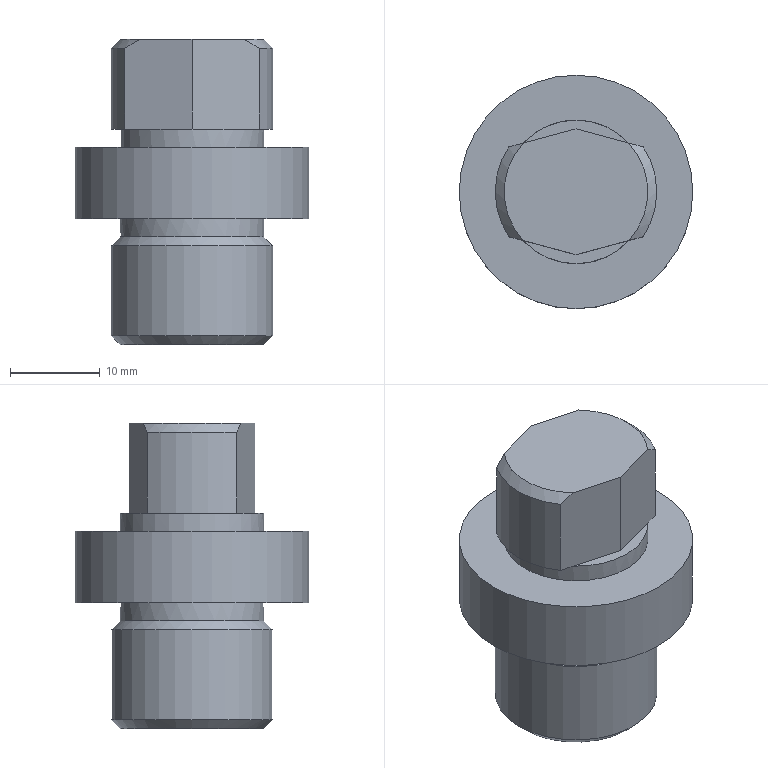Component | NX | DIAMOND_PIN | 1 solid | 22 faces | volume 10042 mm3 | plane 12 | cylinder 6 | cone 4 | commonest cylinder face diameters 18 x3 16 x2 26 x1